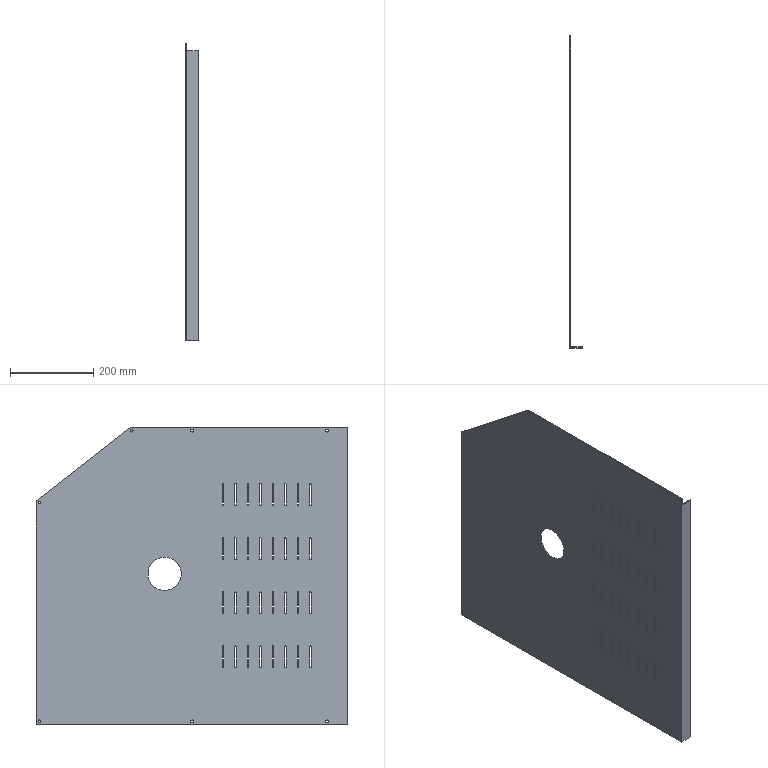Component | SolidWorks | LeftWindow-1 | 1 solid | 186 faces | box 30 x 749 x 715.02 mm | volume 1049385 mm3 | cylinder 112 | plane 74 | commonest cylinder face diameters 3 x96 7 x14 80 x2
build123d program:
from build123d import *

# Parameters (mm, degrees)
BOSS_EXTRUDE1_DEPTH  = 2
SKETCH11_W           = 697.024
SKETCH11_H           = 30
BOSS_EXTRUDE4_DEPTH  = 2
SKETCH12_R           = 40
CUT_EXTRUDE1_DEPTH   = 2
CUT_EXTRUDE2_DEPTH   = 2
LPATTERN1_COUNT      = 4
LPATTERN1_PITCH      = 130
LPATTERN1_COUNT_DIR2 = 8
LPATTERN1_PITCH_DIR2 = 30
SKETCH14_R           = 3.5
CUT_EXTRUDE3_DEPTH   = 2


with BuildPart() as part:
    # Sketch2 → Boss-Extrude1 (new body)
    with BuildSketch(Plane.XY):
        Polygon((-526.457, -703.079), (-526.457, 45.921), (11.543, 45.921), (188.566, -180.659), (188.566, -703.079), align=None)
    extrude(amount=BOSS_EXTRUDE1_DEPTH)

    # Sketch11 → Boss-Extrude4 (add)
    with BuildSketch(Plane(origin=(0, -703.079, 0), x_dir=(-1, 0, 0), z_dir=(0, -1, 0))):
        with Locations((177.945, 13)):
            Rectangle(SKETCH11_W, SKETCH11_H)
    extrude(amount=-BOSS_EXTRUDE4_DEPTH)

    # Sketch12 → Cut-Extrude1 (cut)
    with BuildSketch(Plane.XY.offset(2)):
        with Locations((-163.657, -262.549)):
            Circle(SKETCH12_R)
    extrude(amount=-CUT_EXTRUDE1_DEPTH, mode=Mode.SUBTRACT)

    # Sketch13 → Cut-Extrude2 (cut)
    with BuildSketch(Plane.XY.offset(2)):
        with BuildLine():
            Line((-388.457, -401.579), (-338.457, -401.579))
            ThreePointArc((-338.457, -401.579), (-336.957, -403.079), (-338.457, -404.579))
            Line((-338.457, -404.579), (-388.457, -404.579))
            ThreePointArc((-388.457, -404.579), (-389.957, -403.079), (-388.457, -401.579))
        make_face()
    cut_extrude2 = extrude(amount=-CUT_EXTRUDE2_DEPTH, mode=Mode.SUBTRACT)

    # LPattern1: Cut-Extrude2 4 × 8
    with Locations(*[(i * LPATTERN1_PITCH, -j * LPATTERN1_PITCH_DIR2, 0) for i in range(LPATTERN1_COUNT) for j in range(LPATTERN1_COUNT_DIR2) if (i, j) != (0, 0)]):
        add(cut_extrude2, mode=Mode.SUBTRACT)

    # Sketch14 → Cut-Extrude3 (cut)
    with BuildSketch(Plane.XY.offset(2)):
        with Locations((-518.457, 37.921)):
            Circle(SKETCH14_R)
        with Locations((-518.457, -328.579)):
            Circle(SKETCH14_R)
        with Locations((-518.457, -653.079)):
            Circle(SKETCH14_R)
        with Locations((7.641, 37.921)):
            Circle(SKETCH14_R)
        with Locations((180.566, -183.414)):
            Circle(SKETCH14_R)
        with Locations((180.566, -328.579)):
            Circle(SKETCH14_R)
        with Locations((180.566, -653.079)):
            Circle(SKETCH14_R)
    extrude(amount=-CUT_EXTRUDE3_DEPTH, mode=Mode.SUBTRACT)


solid = part.part

# Placed as in the assembly
solid = solid.moved(Location((-932.55, 184.645, 221.914), (0, -90, 0)))